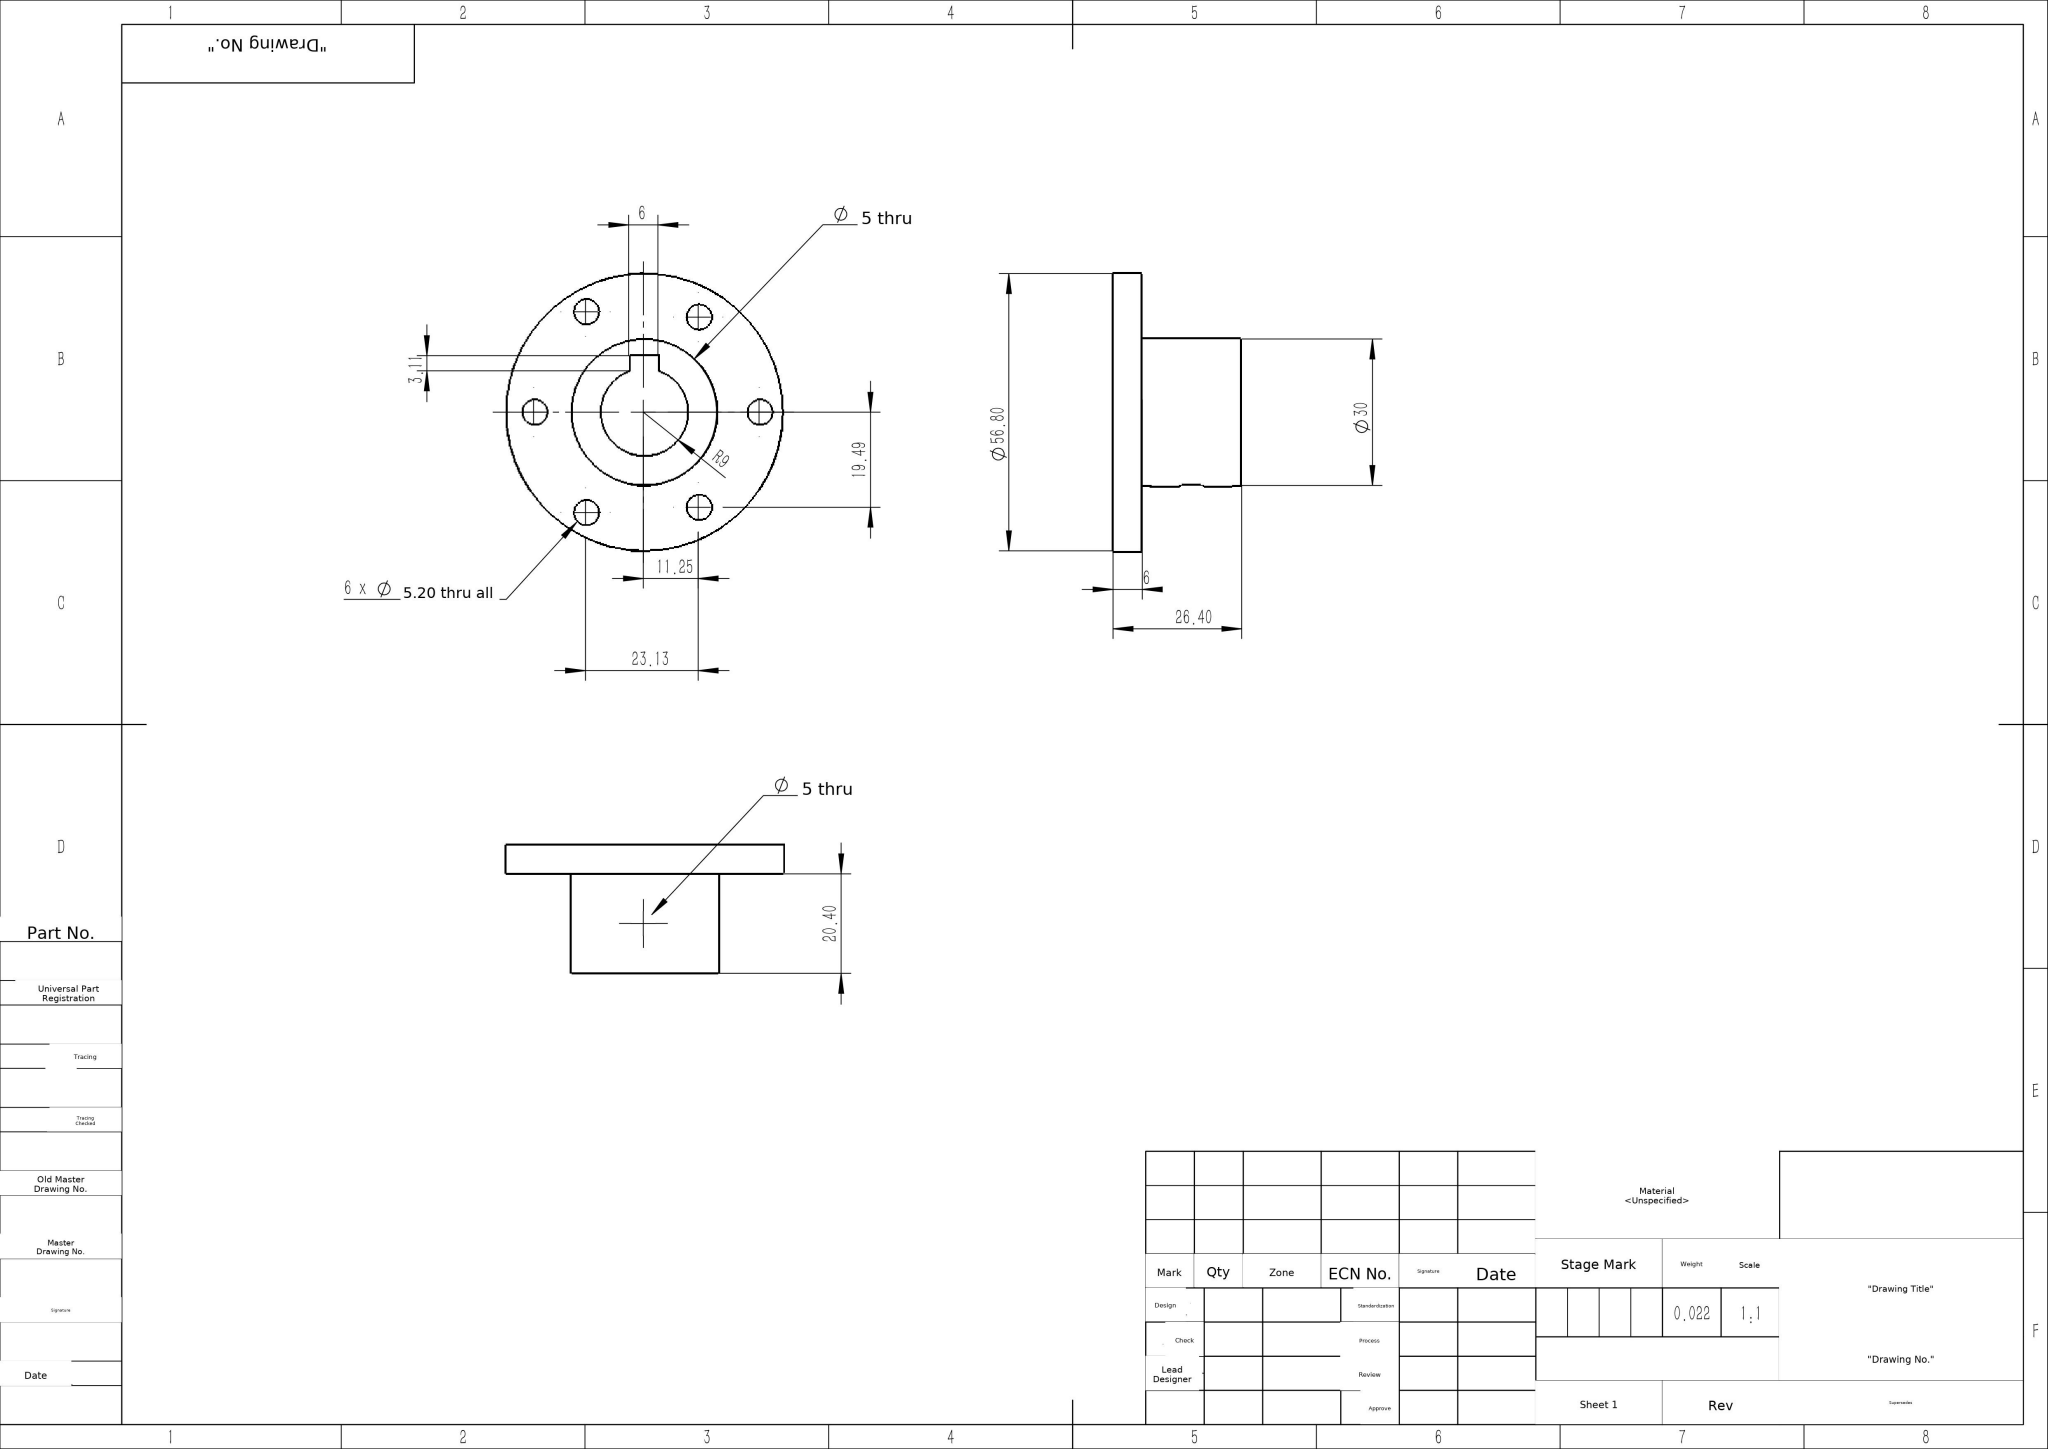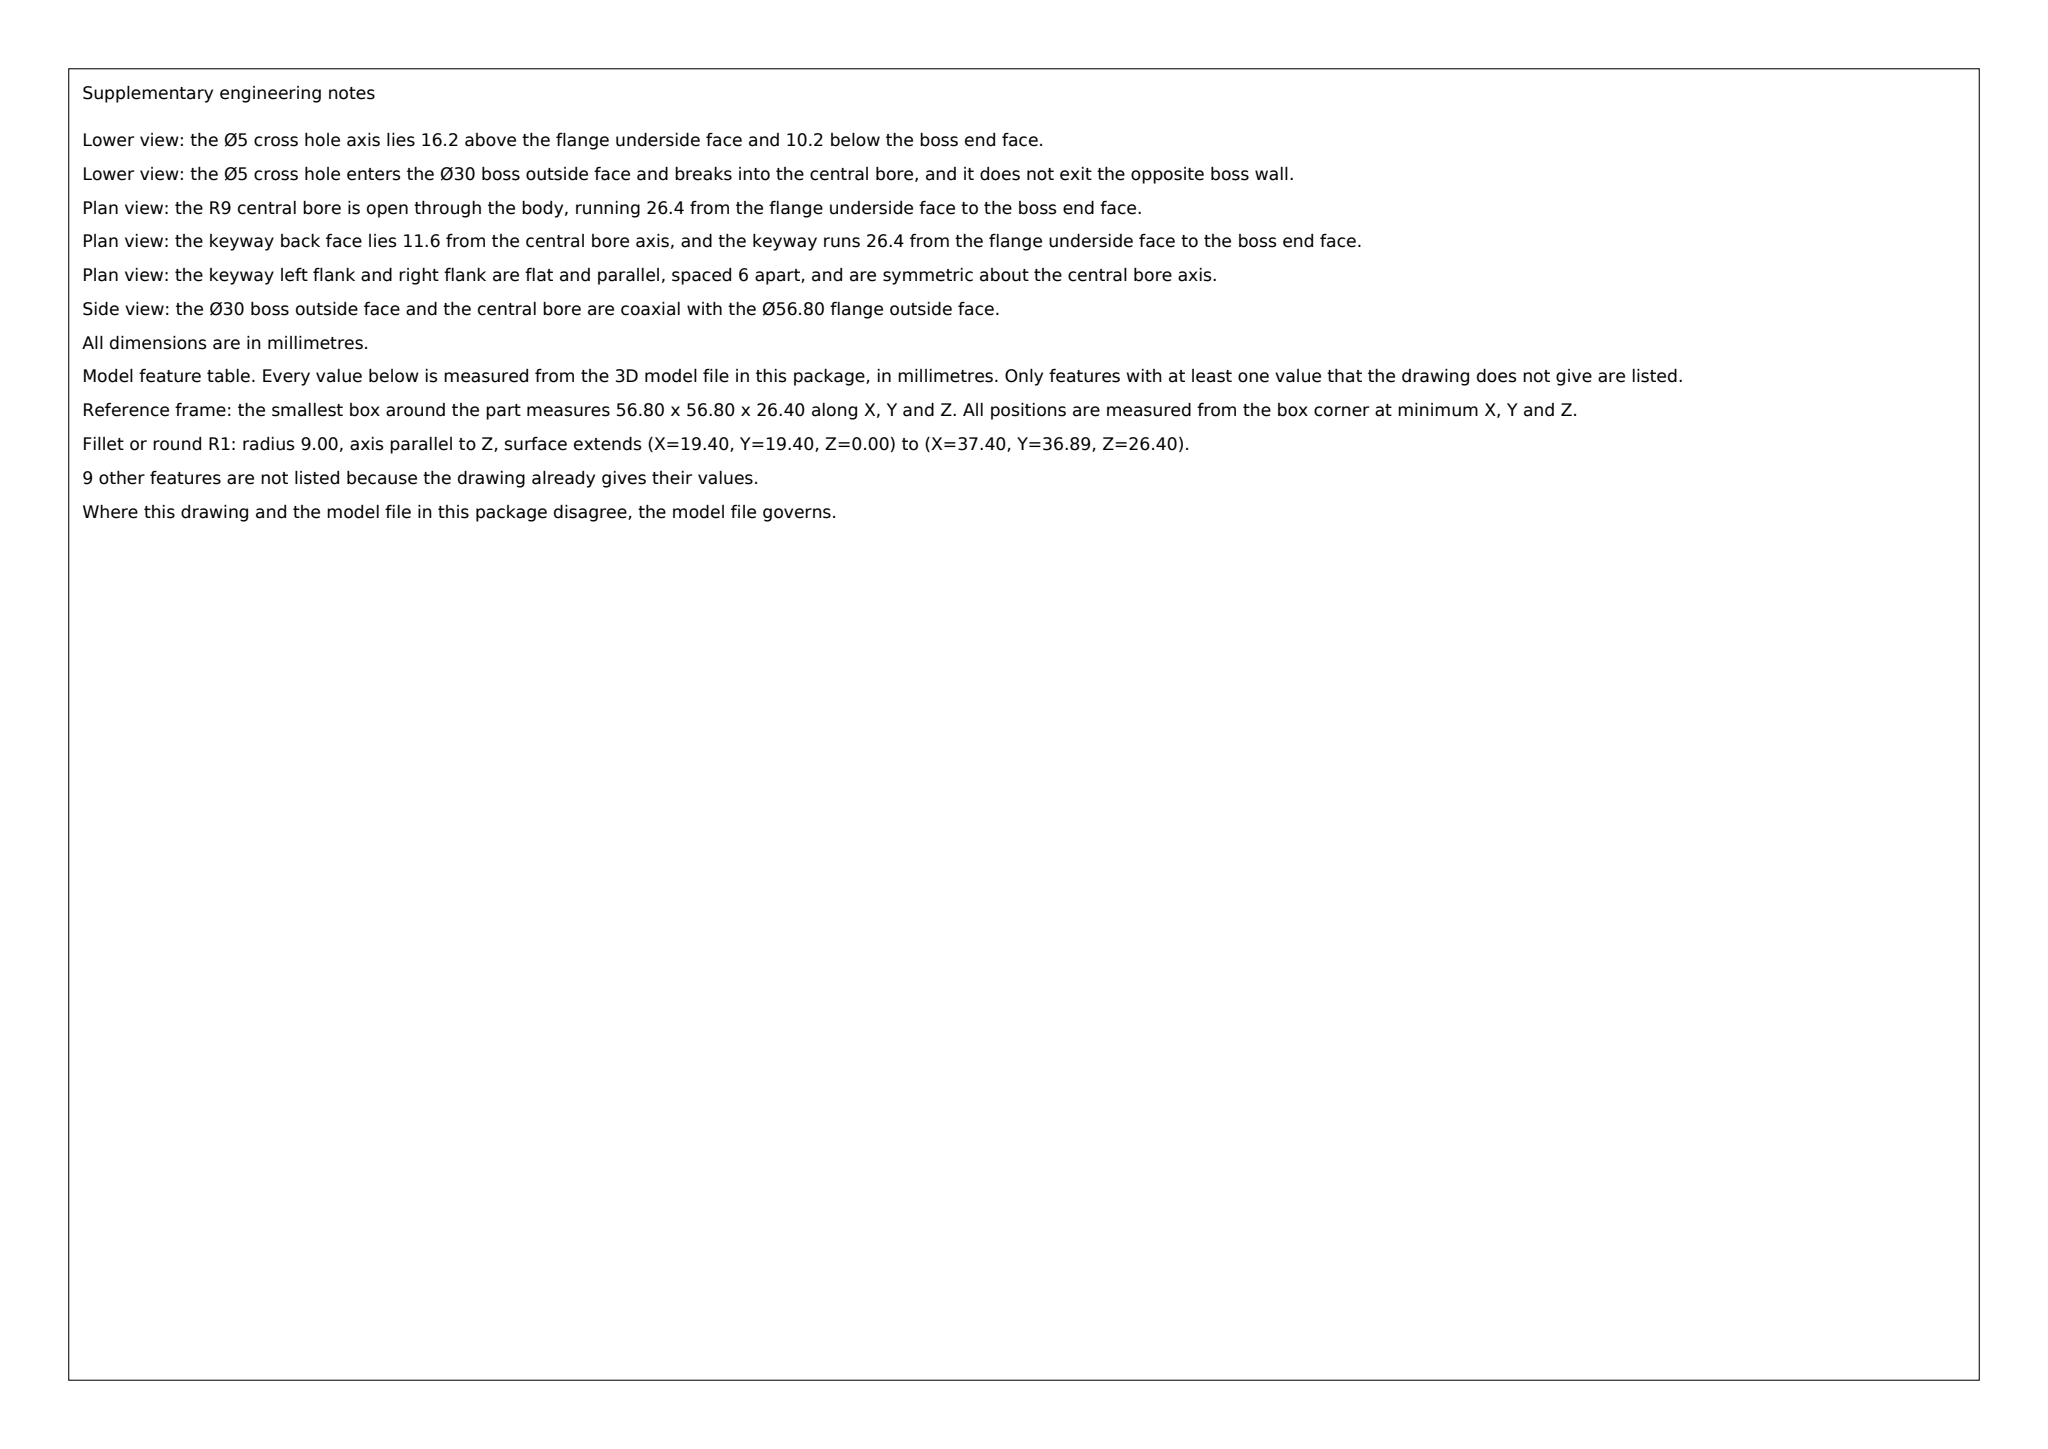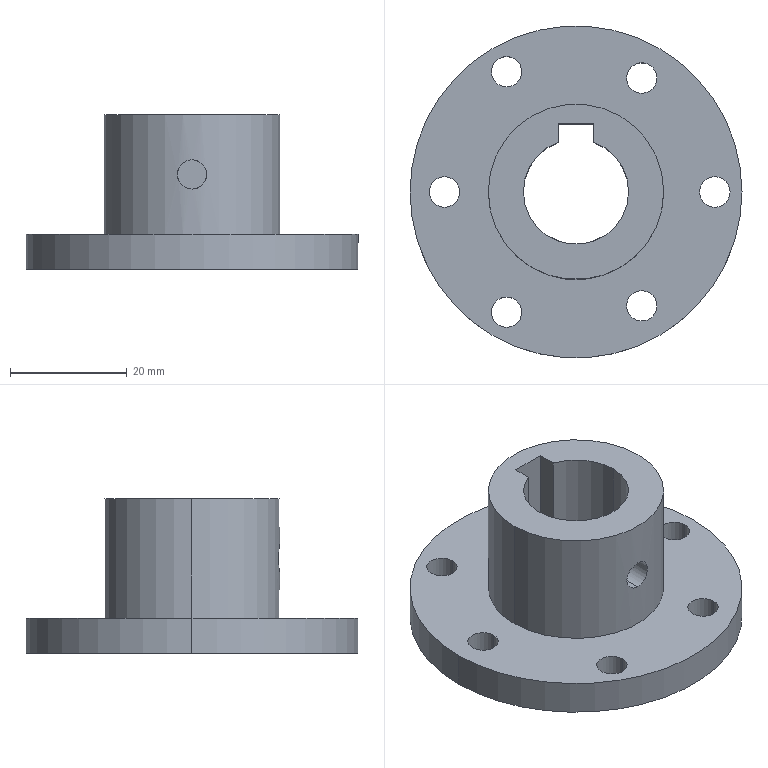Part | SolidWorks | mm | 1 solid | 27 faces | box 56.8 x 56.8 x 26.4 mm | volume 21583 mm3 | cylinder 21 | plane 6 | commonest cylinder face diameters 5.2 x12 18 x3 5 x2 30 x2 56.8 x2
build123d program:
from build123d import *

# Parameters (mm, degrees)
SKETCH1_W                      = 28.4
SKETCH1_H                      = 6
SKETCH2_R                      = 15
BOSS_EXTRUDE1_DEPTH            = 20.4
CUT_EXTRUDE1_DEPTH             = 49.063
SKETCH4_W                      = 9
SKETCH4_H                      = 26.4
F_5_2_5_2_DIAMETER_HOLE1_D     = 5.2
F_5_2_5_2_DIAMETER_HOLE1_DEPTH = 26.4
F_5_0_5_DIAMETER_HOLE1_REACH   = 56.337
F_5_0_5_DIAMETER_HOLE1_BORE_R  = 2.5


with BuildPart() as part:
    # Sketch1 → Revolve1 (revolve)
    with BuildSketch(Plane(origin=(0, 0, 0), x_dir=(1, 0, 0), z_dir=(0, 1, 0))):
        with Locations((14.2, -3)):
            Rectangle(SKETCH1_W, SKETCH1_H)
    revolve(axis=Axis((0, 0, 0), (0, 0, 1)))

    # Sketch2 → Boss-Extrude1 (add)
    with BuildSketch(Plane.XY.offset(6)):
        Circle(SKETCH2_R)
    extrude(amount=BOSS_EXTRUDE1_DEPTH)

    # Sketch3 → Cut-Extrude1 (cut, through all)
    with BuildSketch(Plane(origin=(0, 0, 0), x_dir=(-1, 0, 0), z_dir=(0, 0, -1))):
        with BuildLine():
            Line((3, 11.6), (-3, 11.6))
            Line((-3, 11.6), (-3, 8.485))
            ThreePointArc((-3, 8.485), (0, 9), (3, 8.485))
            Line((3, 8.485), (3, 11.6))
        make_face()
    extrude(amount=-CUT_EXTRUDE1_DEPTH, mode=Mode.SUBTRACT)

    # Sketch4 → Cut-Revolve1 (revolve, cut)
    with BuildSketch(Plane(origin=(0, 0, 0), x_dir=(1, 0, 0), z_dir=(0, 1, 0))):
        with Locations((4.5, -13.2)):
            Rectangle(SKETCH4_W, SKETCH4_H)
    revolve(axis=Axis((0, 0, 0), (0, 0, 1)), mode=Mode.SUBTRACT)

    # 5.2 _5.2_ Diameter Hole1
    with Locations(Plane(origin=(0, 0, 0), x_dir=(-1, 0, 0), z_dir=(0, 0, -1))):
        with Locations((11.875, -20.568), (-23.75, 0), (-11.25, -19.486), (22.5, 0), (-11.25, 19.486), (11.875, 20.568)):
            Hole(F_5_2_5_2_DIAMETER_HOLE1_D / 2, depth=F_5_2_5_2_DIAMETER_HOLE1_DEPTH)

    # 5.0 _5_ Diameter Hole1 bore (on position points) → 5.0 _5_ Diameter Hole1 (cut, up to next)
    with BuildSketch(Plane(origin=(0, -15, 16.2), x_dir=(-1, 0, 0), z_dir=(0, -1, 0)), mode=Mode.PRIVATE) as f_5_0_5_diameter_hole1_sk1:
        Circle(F_5_0_5_DIAMETER_HOLE1_BORE_R)
    f_5_0_5_diameter_hole1_tool1 = extrude(f_5_0_5_diameter_hole1_sk1.sketch, amount=-F_5_0_5_DIAMETER_HOLE1_REACH, mode=Mode.PRIVATE) & part.part
    add(f_5_0_5_diameter_hole1_tool1.solids().sort_by_distance((0, -15, 16.2))[0], mode=Mode.SUBTRACT)


solid = part.part